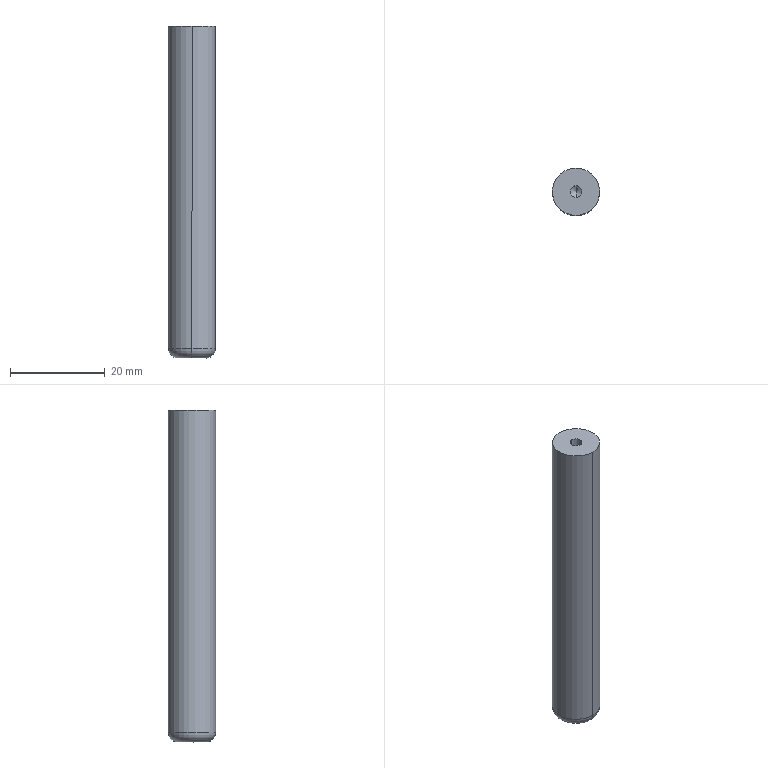Component | SolidWorks | 2SZT-2-010-1 | 1 solid | 10 faces | box 10 x 10 x 70 mm | volume 5435 mm3 | cylinder 4 | cone 2 | torus 2 | plane 2 | commonest cylinder face diameters 2.5 x2 10 x2
build123d program:
from build123d import *

# Parameters (mm, degrees)
SKETCH1_R             = 5
BOSS_EXTRUDE1_DEPTH   = 70
FILLET1_R             = 2
M3_TAPPED_HOLE1_D     = 2.5
M3_TAPPED_HOLE1_DEPTH = 7.5
M3_TAPPED_HOLE1_TIP   = 0.7511


with BuildPart() as part:
    # Sketch1 → Boss-Extrude1 (new body)
    with BuildSketch(Plane(origin=(0, 0, 0), x_dir=(1, 0, 0), z_dir=(0, 1, 0))):
        with Locations(Location((0, 0, 0), (0, 0, 270))):
            Circle(SKETCH1_R)
    extrude(amount=BOSS_EXTRUDE1_DEPTH)

    # Fillet1
    fillet1_edges = [part.edges().sort_by_distance(p)[0] for p in [
        (0, 70, -5),
    ]]
    fillet(fillet1_edges, radius=FILLET1_R)

    # M3 Tapped Hole1
    with Locations(Plane(origin=(0, 0, 0), x_dir=(-1, 0, 0), z_dir=(0, -1, 0))):
        with Locations((0, 0)):
            Hole(M3_TAPPED_HOLE1_D / 2, depth=M3_TAPPED_HOLE1_DEPTH)
            with Locations((0, 0, -(M3_TAPPED_HOLE1_DEPTH + M3_TAPPED_HOLE1_TIP / 2))):  # 118° drill point
                Cone(0, M3_TAPPED_HOLE1_D / 2, M3_TAPPED_HOLE1_TIP, mode=Mode.SUBTRACT)


solid = part.part

# Placed as in the assembly
solid = solid.moved(Location((1000.265, 375.193, -286.266), (-90, 0, 0)))
STEP:
#1=CARTESIAN_POINT('',(39.381,14.821,-11.566));
#2=VERTEX_POINT('',#1);
#3=CARTESIAN_POINT('',(39.381,14.722,-11.566));
#4=VERTEX_POINT('',#3);
#5=CARTESIAN_POINT('',(39.381,14.771,-11.566));
#6=DIRECTION('',(0.00002551,0.,1.));
#7=DIRECTION('',(0.00002551,-1.,-0.));
#8=AXIS2_PLACEMENT_3D('',#5,#6,#7);
#9=CIRCLE('',#8,0.04921);
#10=EDGE_CURVE('',#2,#4,#9,.T.);
#11=ORIENTED_EDGE('',*,*,#10,.F.);
#12=CARTESIAN_POINT('',(39.381,14.821,-11.27));
#13=VERTEX_POINT('',#12);
#14=CARTESIAN_POINT('',(39.381,14.821,-11.27));
#15=DIRECTION('',(0.00002551,0.,1.));
#16=VECTOR('',#15,39.37);
#17=LINE('',#14,#16);
#18=EDGE_CURVE('',#2,#13,#17,.T.);
#19=ORIENTED_EDGE('',*,*,#18,.T.);
#20=CARTESIAN_POINT('',(39.381,14.722,-11.27));
#21=VERTEX_POINT('',#20);
#22=CARTESIAN_POINT('',(39.381,14.771,-11.27));
#23=DIRECTION('',(0.00002551,0.,1.));
#24=DIRECTION('',(0.00002551,-1.,-0.));
#25=AXIS2_PLACEMENT_3D('',#22,#23,#24);
#26=CIRCLE('',#25,0.04921);
#27=EDGE_CURVE('',#13,#21,#26,.T.);
#28=ORIENTED_EDGE('',*,*,#27,.T.);
#29=CARTESIAN_POINT('',(39.381,14.722,-11.27));
#30=DIRECTION('',(0.00002551,0.,1.));
#31=VECTOR('',#30,39.37);
#32=LINE('',#29,#31);
#33=EDGE_CURVE('',#4,#21,#32,.T.);
#34=ORIENTED_EDGE('',*,*,#33,.F.);
#35=EDGE_LOOP('',(#11,#19,#28,#34));
#36=FACE_OUTER_BOUND('',#35,.T.);
#37=CARTESIAN_POINT('',(39.381,14.771,-11.27));
#38=DIRECTION('',(0.00002551,0.,1.));
#39=DIRECTION('',(0.00002551,-1.,-0.));
#40=AXIS2_PLACEMENT_3D('',#37,#38,#39);
#41=CYLINDRICAL_SURFACE('',#40,0.04921);
#42=ADVANCED_FACE('',(#36),#41,.F.);
#43=CARTESIAN_POINT('',(39.381,14.771,-11.595));
#44=VERTEX_POINT('',#43);
#45=CARTESIAN_POINT('',(39.381,14.722,-11.566));
#46=DIRECTION('',(0.000035,-0.8572,0.515));
#47=VECTOR('',#46,39.37);
#48=LINE('',#45,#47);
#49=EDGE_CURVE('',#44,#4,#48,.T.);
#50=ORIENTED_EDGE('',*,*,#49,.F.);
#51=CARTESIAN_POINT('',(39.381,14.821,-11.566));
#52=DIRECTION('',(-0.00000873,0.8572,0.515));
#53=VECTOR('',#52,39.37);
#54=LINE('',#51,#53);
#55=EDGE_CURVE('',#44,#2,#54,.T.);
#56=ORIENTED_EDGE('',*,*,#55,.T.);
#57=ORIENTED_EDGE('',*,*,#10,.T.);
#58=EDGE_LOOP('',(#50,#56,#57));
#59=FACE_OUTER_BOUND('',#58,.T.);
#60=CARTESIAN_POINT('',(39.381,14.771,-11.566));
#61=DIRECTION('',(0.00002551,0.,1.));
#62=DIRECTION('',(0.00002551,-1.,-0.));
#63=AXIS2_PLACEMENT_3D('',#60,#61,#62);
#64=CONICAL_SURFACE('',#63,0.04921,1.03);
#65=ADVANCED_FACE('',(#59),#64,.F.);
#66=CARTESIAN_POINT('',(39.38,14.575,-13.947));
#67=VERTEX_POINT('',#66);
#68=CARTESIAN_POINT('',(39.38,14.968,-13.947));
#69=VERTEX_POINT('',#68);
#70=CARTESIAN_POINT('',(39.38,14.771,-13.947));
#71=DIRECTION('',(0.00002551,0.,1.));
#72=DIRECTION('',(-0.00002551,1.,0.));
#73=AXIS2_PLACEMENT_3D('',#70,#71,#72);
#74=CIRCLE('',#73,0.1969);
#75=EDGE_CURVE('',#67,#69,#74,.T.);
#76=ORIENTED_EDGE('',*,*,#75,.F.);
#77=CARTESIAN_POINT('',(39.38,14.653,-14.026));
#78=VERTEX_POINT('',#77);
#79=CARTESIAN_POINT('',(39.38,14.653,-13.947));
#80=DIRECTION('',(1.,0.00002551,-0.00002551));
#81=DIRECTION('',(-0.00002551,1.,0.));
#82=AXIS2_PLACEMENT_3D('',#79,#80,#81);
#83=CIRCLE('',#82,0.07874);
#84=EDGE_CURVE('',#67,#78,#83,.T.);
#85=ORIENTED_EDGE('',*,*,#84,.T.);
#86=CARTESIAN_POINT('',(39.38,14.889,-14.026));
#87=VERTEX_POINT('',#86);
#88=CARTESIAN_POINT('',(39.38,14.771,-14.026));
#89=DIRECTION('',(-0.00002551,-0.,-1.));
#90=DIRECTION('',(-0.00002551,1.,0.));
#91=AXIS2_PLACEMENT_3D('',#88,#89,#90);
#92=CIRCLE('',#91,0.1181);
#93=EDGE_CURVE('',#87,#78,#92,.T.);
#94=ORIENTED_EDGE('',*,*,#93,.F.);
#95=CARTESIAN_POINT('',(39.38,14.889,-13.947));
#96=DIRECTION('',(-1.,-0.00002551,0.00002551));
#97=DIRECTION('',(0.00002551,-1.,0.));
#98=AXIS2_PLACEMENT_3D('',#95,#96,#97);
#99=CIRCLE('',#98,0.07874);
#100=EDGE_CURVE('',#69,#87,#99,.T.);
#101=ORIENTED_EDGE('',*,*,#100,.F.);
#102=EDGE_LOOP('',(#76,#85,#94,#101));
#103=FACE_OUTER_BOUND('',#102,.T.);
#104=CARTESIAN_POINT('',(39.38,14.771,-13.947));
#105=DIRECTION('',(-0.00002551,-0.,-1.));
#106=DIRECTION('',(-0.00002551,1.,0.));
#107=AXIS2_PLACEMENT_3D('',#104,#105,#106);
#108=TOROIDAL_SURFACE('',#107,0.1181,0.07874);
#109=ADVANCED_FACE('',(#103),#108,.T.);
#110=ORIENTED_EDGE('',*,*,#75,.T.);
#111=CARTESIAN_POINT('',(39.381,14.968,-11.27));
#112=VERTEX_POINT('',#111);
#113=CARTESIAN_POINT('',(39.38,14.968,-14.026));
#114=DIRECTION('',(0.00002551,0.,1.));
#115=VECTOR('',#114,39.37);
#116=LINE('',#113,#115);
#117=EDGE_CURVE('',#69,#112,#116,.T.);
#118=ORIENTED_EDGE('',*,*,#117,.T.);
#119=CARTESIAN_POINT('',(39.381,14.575,-11.27));
#120=VERTEX_POINT('',#119);
#121=CARTESIAN_POINT('',(39.381,14.771,-11.27));
#122=DIRECTION('',(-0.00002551,-0.,-1.));
#123=DIRECTION('',(-0.00002551,1.,0.));
#124=AXIS2_PLACEMENT_3D('',#121,#122,#123);
#125=CIRCLE('',#124,0.1969);
#126=EDGE_CURVE('',#112,#120,#125,.T.);
#127=ORIENTED_EDGE('',*,*,#126,.T.);
#128=CARTESIAN_POINT('',(39.38,14.575,-14.026));
#129=DIRECTION('',(0.00002551,0.,1.));
#130=VECTOR('',#129,39.37);
#131=LINE('',#128,#130);
#132=EDGE_CURVE('',#67,#120,#131,.T.);
#133=ORIENTED_EDGE('',*,*,#132,.F.);
#134=EDGE_LOOP('',(#110,#118,#127,#133));
#135=FACE_OUTER_BOUND('',#134,.T.);
#136=CARTESIAN_POINT('',(39.38,14.771,-14.026));
#137=DIRECTION('',(0.00002551,0.,1.));
#138=DIRECTION('',(0.00002551,-1.,-0.));
#139=AXIS2_PLACEMENT_3D('',#136,#137,#138);
#140=CYLINDRICAL_SURFACE('',#139,0.1969);
#141=ADVANCED_FACE('',(#135),#140,.T.);
#142=ORIENTED_EDGE('',*,*,#117,.F.);
#143=CARTESIAN_POINT('',(39.38,14.771,-13.947));
#144=DIRECTION('',(0.00002551,0.,1.));
#145=DIRECTION('',(-0.00002551,1.,0.));
#146=AXIS2_PLACEMENT_3D('',#143,#144,#145);
#147=CIRCLE('',#146,0.1969);
#148=EDGE_CURVE('',#69,#67,#147,.T.);
#149=ORIENTED_EDGE('',*,*,#148,.T.);
#150=ORIENTED_EDGE('',*,*,#132,.T.);
#151=CARTESIAN_POINT('',(39.381,14.771,-11.27));
#152=DIRECTION('',(-0.00002551,-0.,-1.));
#153=DIRECTION('',(-0.00002551,1.,0.));
#154=AXIS2_PLACEMENT_3D('',#151,#152,#153);
#155=CIRCLE('',#154,0.1969);
#156=EDGE_CURVE('',#120,#112,#155,.T.);
#157=ORIENTED_EDGE('',*,*,#156,.T.);
#158=EDGE_LOOP('',(#142,#149,#150,#157));
#159=FACE_OUTER_BOUND('',#158,.T.);
#160=CARTESIAN_POINT('',(39.38,14.771,-14.026));
#161=DIRECTION('',(0.00002551,0.,1.));
#162=DIRECTION('',(0.00002551,-1.,-0.));
#163=AXIS2_PLACEMENT_3D('',#160,#161,#162);
#164=CYLINDRICAL_SURFACE('',#163,0.1969);
#165=ADVANCED_FACE('',(#159),#164,.T.);
#166=ORIENTED_EDGE('',*,*,#93,.T.);
#167=CARTESIAN_POINT('',(39.38,14.771,-14.026));
#168=DIRECTION('',(-0.00002551,-0.,-1.));
#169=DIRECTION('',(-0.00002551,1.,0.));
#170=AXIS2_PLACEMENT_3D('',#167,#168,#169);
#171=CIRCLE('',#170,0.1181);
#172=EDGE_CURVE('',#78,#87,#171,.T.);
#173=ORIENTED_EDGE('',*,*,#172,.T.);
#174=EDGE_LOOP('',(#166,#173));
#175=FACE_OUTER_BOUND('',#174,.T.);
#176=CARTESIAN_POINT('',(39.38,14.771,-14.026));
#177=DIRECTION('',(-0.00002551,-0.,-1.));
#178=DIRECTION('',(-0.00002551,1.,0.));
#179=AXIS2_PLACEMENT_3D('',#176,#177,#178);
#180=PLANE('',#179);
#181=ADVANCED_FACE('',(#175),#180,.T.);
#182=CARTESIAN_POINT('',(39.381,14.771,-11.27));
#183=DIRECTION('',(0.00002551,0.,1.));
#184=DIRECTION('',(0.00002551,-1.,-0.));
#185=AXIS2_PLACEMENT_3D('',#182,#183,#184);
#186=CIRCLE('',#185,0.04921);
#187=EDGE_CURVE('',#21,#13,#186,.T.);
#188=ORIENTED_EDGE('',*,*,#187,.F.);
#189=ORIENTED_EDGE('',*,*,#27,.F.);
#190=EDGE_LOOP('',(#188,#189));
#191=FACE_BOUND('',#190,.T.);
#192=ORIENTED_EDGE('',*,*,#156,.F.);
#193=ORIENTED_EDGE('',*,*,#126,.F.);
#194=EDGE_LOOP('',(#192,#193));
#195=FACE_OUTER_BOUND('',#194,.T.);
#196=CARTESIAN_POINT('',(39.381,14.771,-11.27));
#197=DIRECTION('',(-0.00002551,-0.,-1.));
#198=DIRECTION('',(-0.00002551,1.,0.));
#199=AXIS2_PLACEMENT_3D('',#196,#197,#198);
#200=PLANE('',#199);
#201=ADVANCED_FACE('',(#191,#195),#200,.F.);
#202=ORIENTED_EDGE('',*,*,#84,.F.);
#203=ORIENTED_EDGE('',*,*,#148,.F.);
#204=ORIENTED_EDGE('',*,*,#100,.T.);
#205=ORIENTED_EDGE('',*,*,#172,.F.);
#206=EDGE_LOOP('',(#202,#203,#204,#205));
#207=FACE_OUTER_BOUND('',#206,.T.);
#208=CARTESIAN_POINT('',(39.38,14.771,-13.947));
#209=DIRECTION('',(-0.00002551,-0.,-1.));
#210=DIRECTION('',(-0.00002551,1.,0.));
#211=AXIS2_PLACEMENT_3D('',#208,#209,#210);
#212=TOROIDAL_SURFACE('',#211,0.1181,0.07874);
#213=ADVANCED_FACE('',(#207),#212,.T.);
#214=ORIENTED_EDGE('',*,*,#55,.F.);
#215=ORIENTED_EDGE('',*,*,#49,.T.);
#216=CARTESIAN_POINT('',(39.381,14.771,-11.566));
#217=DIRECTION('',(0.00002551,0.,1.));
#218=DIRECTION('',(0.00002551,-1.,-0.));
#219=AXIS2_PLACEMENT_3D('',#216,#217,#218);
#220=CIRCLE('',#219,0.04921);
#221=EDGE_CURVE('',#4,#2,#220,.T.);
#222=ORIENTED_EDGE('',*,*,#221,.T.);
#223=EDGE_LOOP('',(#214,#215,#222));
#224=FACE_OUTER_BOUND('',#223,.T.);
#225=CARTESIAN_POINT('',(39.381,14.771,-11.566));
#226=DIRECTION('',(0.00002551,0.,1.));
#227=DIRECTION('',(0.00002551,-1.,-0.));
#228=AXIS2_PLACEMENT_3D('',#225,#226,#227);
#229=CONICAL_SURFACE('',#228,0.04921,1.03);
#230=ADVANCED_FACE('',(#224),#229,.F.);
#231=ORIENTED_EDGE('',*,*,#18,.F.);
#232=ORIENTED_EDGE('',*,*,#221,.F.);
#233=ORIENTED_EDGE('',*,*,#33,.T.);
#234=ORIENTED_EDGE('',*,*,#187,.T.);
#235=EDGE_LOOP('',(#231,#232,#233,#234));
#236=FACE_OUTER_BOUND('',#235,.T.);
#237=CARTESIAN_POINT('',(39.381,14.771,-11.27));
#238=DIRECTION('',(0.00002551,0.,1.));
#239=DIRECTION('',(0.00002551,-1.,-0.));
#240=AXIS2_PLACEMENT_3D('',#237,#238,#239);
#241=CYLINDRICAL_SURFACE('',#240,0.04921);
#242=ADVANCED_FACE('',(#236),#241,.F.);
#243=CLOSED_SHELL('',(#42,#65,#109,#141,#165,#181,#201,#213,#230,#242));
#244=MANIFOLD_SOLID_BREP('',#243);
#245=CARTESIAN_POINT('',(0.,0.,0.));
#246=DIRECTION('',(0.,0.,1.));
#247=DIRECTION('',(1.,0.,0.));
#248=AXIS2_PLACEMENT_3D('',#245,#246,#247);
#249=(LENGTH_UNIT()NAMED_UNIT(*)SI_UNIT($,.METRE.));
#250=LENGTH_MEASURE_WITH_UNIT(LENGTH_MEASURE(0.0254),#249);
#251=DIMENSIONAL_EXPONENTS(1.,0.,0.,0.,0.,0.,0.);
#252=(CONVERSION_BASED_UNIT('',#250)LENGTH_UNIT()NAMED_UNIT(#251));
#253=UNCERTAINTY_MEASURE_WITH_UNIT(LENGTH_MEASURE(0.00001),#252,'','');
#254=(NAMED_UNIT(*)PLANE_ANGLE_UNIT()SI_UNIT($,.RADIAN.));
#255=(NAMED_UNIT(*)SI_UNIT($,.STERADIAN.)SOLID_ANGLE_UNIT());
#256=(GEOMETRIC_REPRESENTATION_CONTEXT(3)GLOBAL_UNCERTAINTY_ASSIGNED_CONTEXT((#253))GLOBAL_UNIT_ASSIGNED_CONTEXT((#252,#254,#255))REPRESENTATION_CONTEXT('',''));
#257=ADVANCED_BREP_SHAPE_REPRESENTATION('',(#244,#248),#256);
#258=COLOUR_RGB('',0.7922,0.8196,0.9333);
#259=FILL_AREA_STYLE_COLOUR('',#258);
#260=FILL_AREA_STYLE('',(#259));
#261=SURFACE_STYLE_FILL_AREA(#260);
#262=SURFACE_SIDE_STYLE('',(#261));
#263=SURFACE_STYLE_USAGE(.BOTH.,#262);
#264=PRESENTATION_STYLE_ASSIGNMENT((#263));
#265=STYLED_ITEM('',(#264),#244);
#266=PRESENTATION_LAYER_ASSIGNMENT('','',(#265));
#267=(LENGTH_UNIT()NAMED_UNIT(*)SI_UNIT($,.METRE.));
#268=LENGTH_MEASURE_WITH_UNIT(LENGTH_MEASURE(0.0254),#267);
#269=DIMENSIONAL_EXPONENTS(1.,0.,0.,0.,0.,0.,0.);
#270=(CONVERSION_BASED_UNIT('',#268)LENGTH_UNIT()NAMED_UNIT(#269));
#271=UNCERTAINTY_MEASURE_WITH_UNIT(LENGTH_MEASURE(0.00001),#270,'','');
#272=(NAMED_UNIT(*)PLANE_ANGLE_UNIT()SI_UNIT($,.RADIAN.));
#273=(NAMED_UNIT(*)SI_UNIT($,.STERADIAN.)SOLID_ANGLE_UNIT());
#274=(GEOMETRIC_REPRESENTATION_CONTEXT(3)GLOBAL_UNCERTAINTY_ASSIGNED_CONTEXT((#271))GLOBAL_UNIT_ASSIGNED_CONTEXT((#270,#272,#273))REPRESENTATION_CONTEXT('',''));
#275=MECHANICAL_DESIGN_GEOMETRIC_PRESENTATION_REPRESENTATION('',(#265),#274);